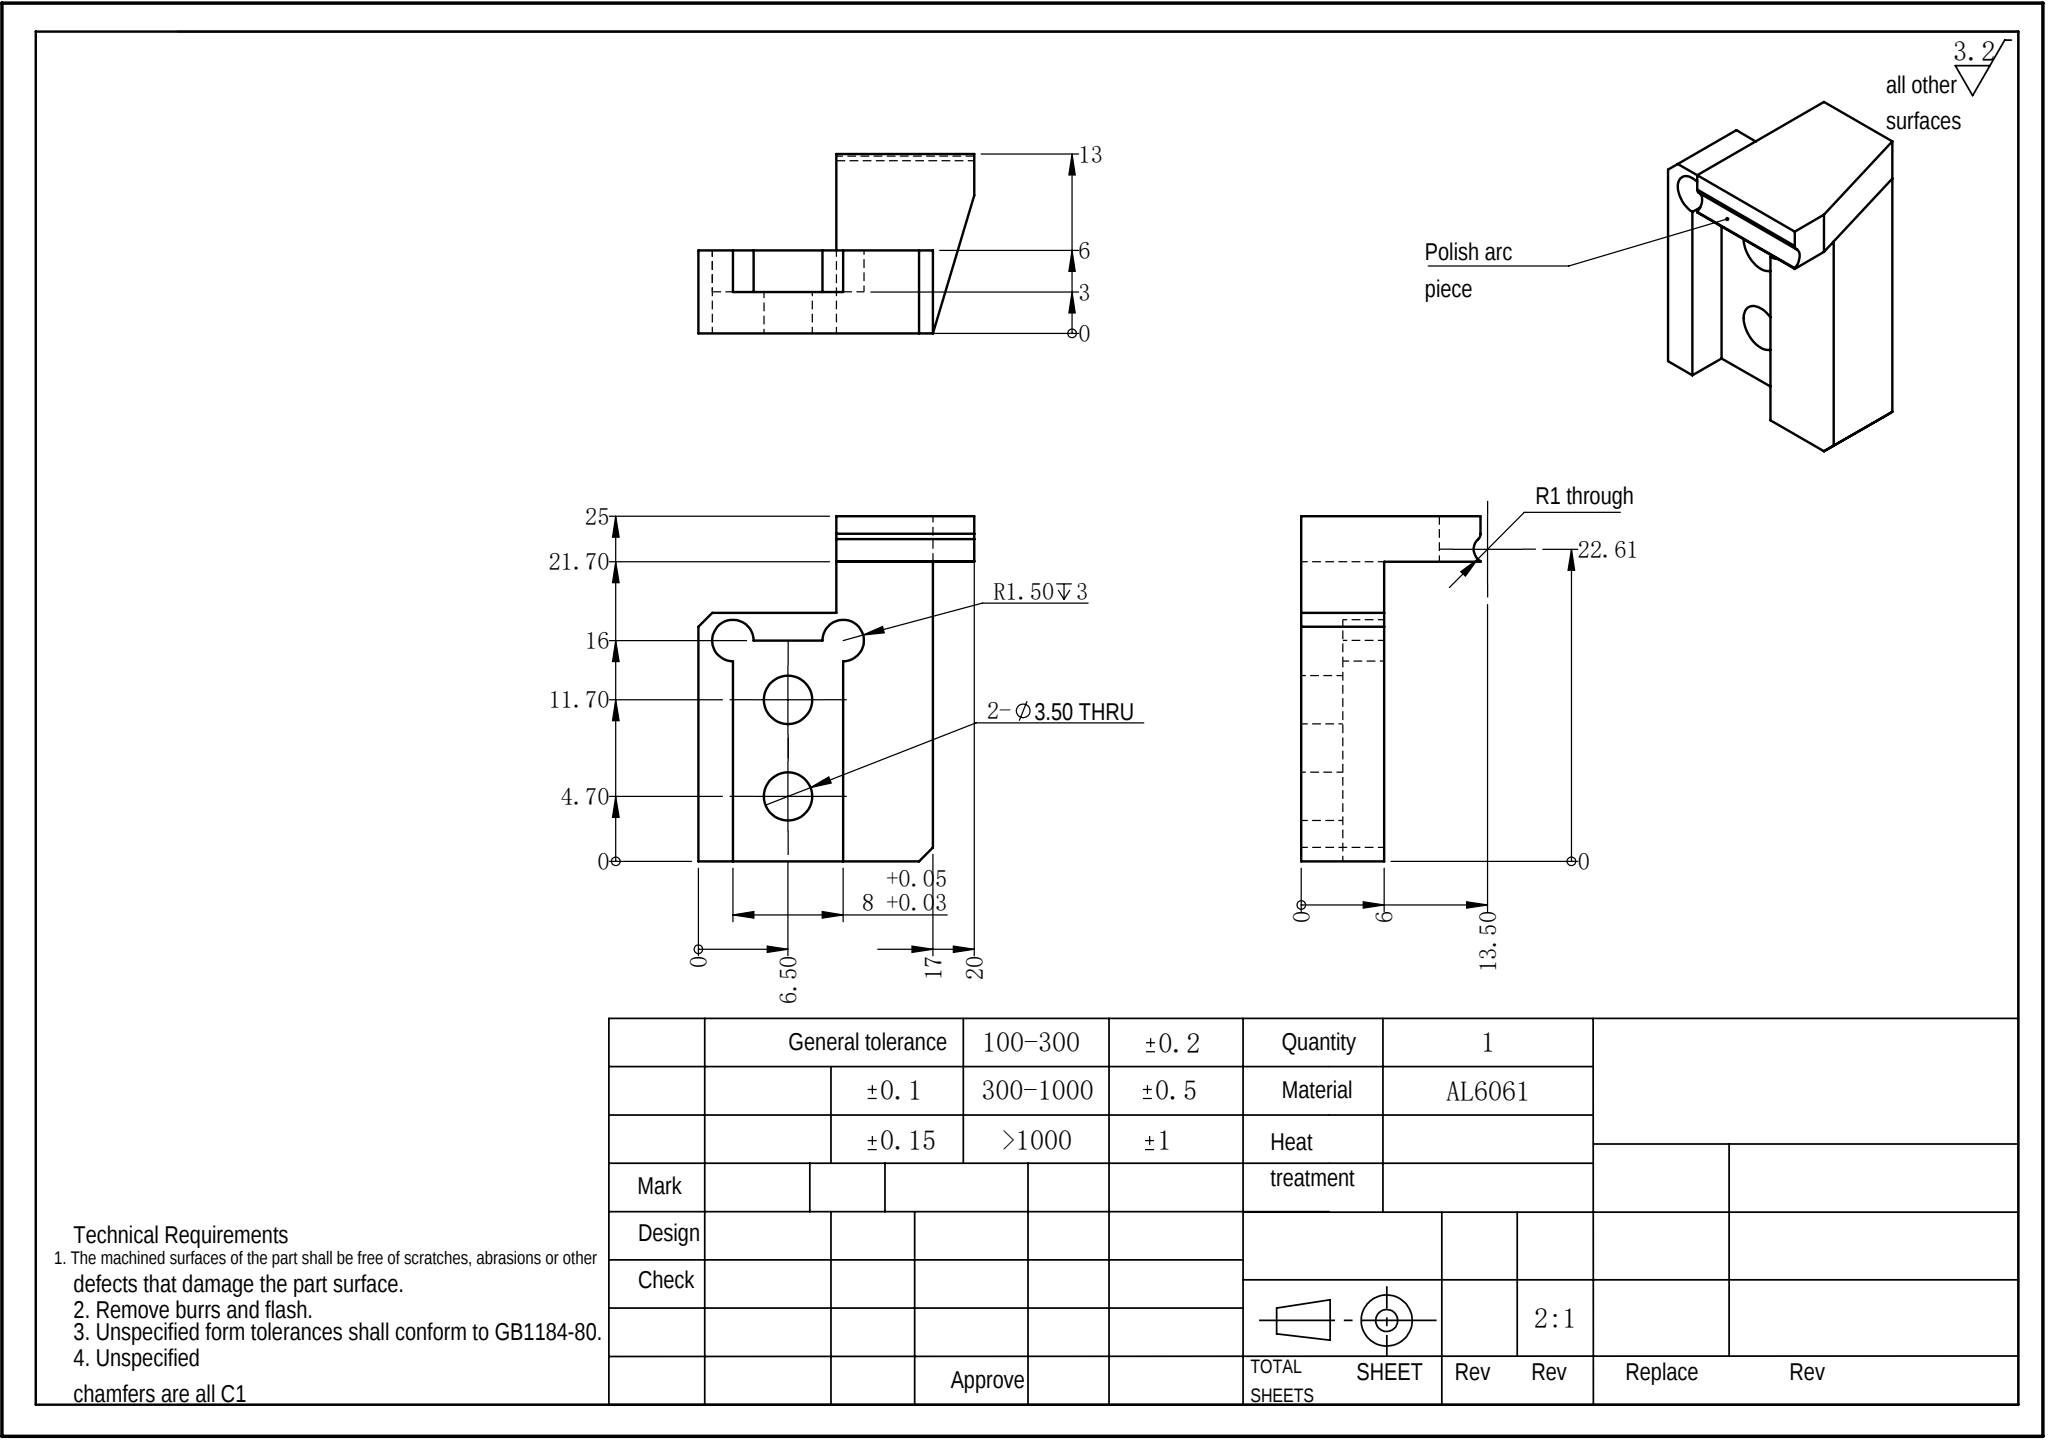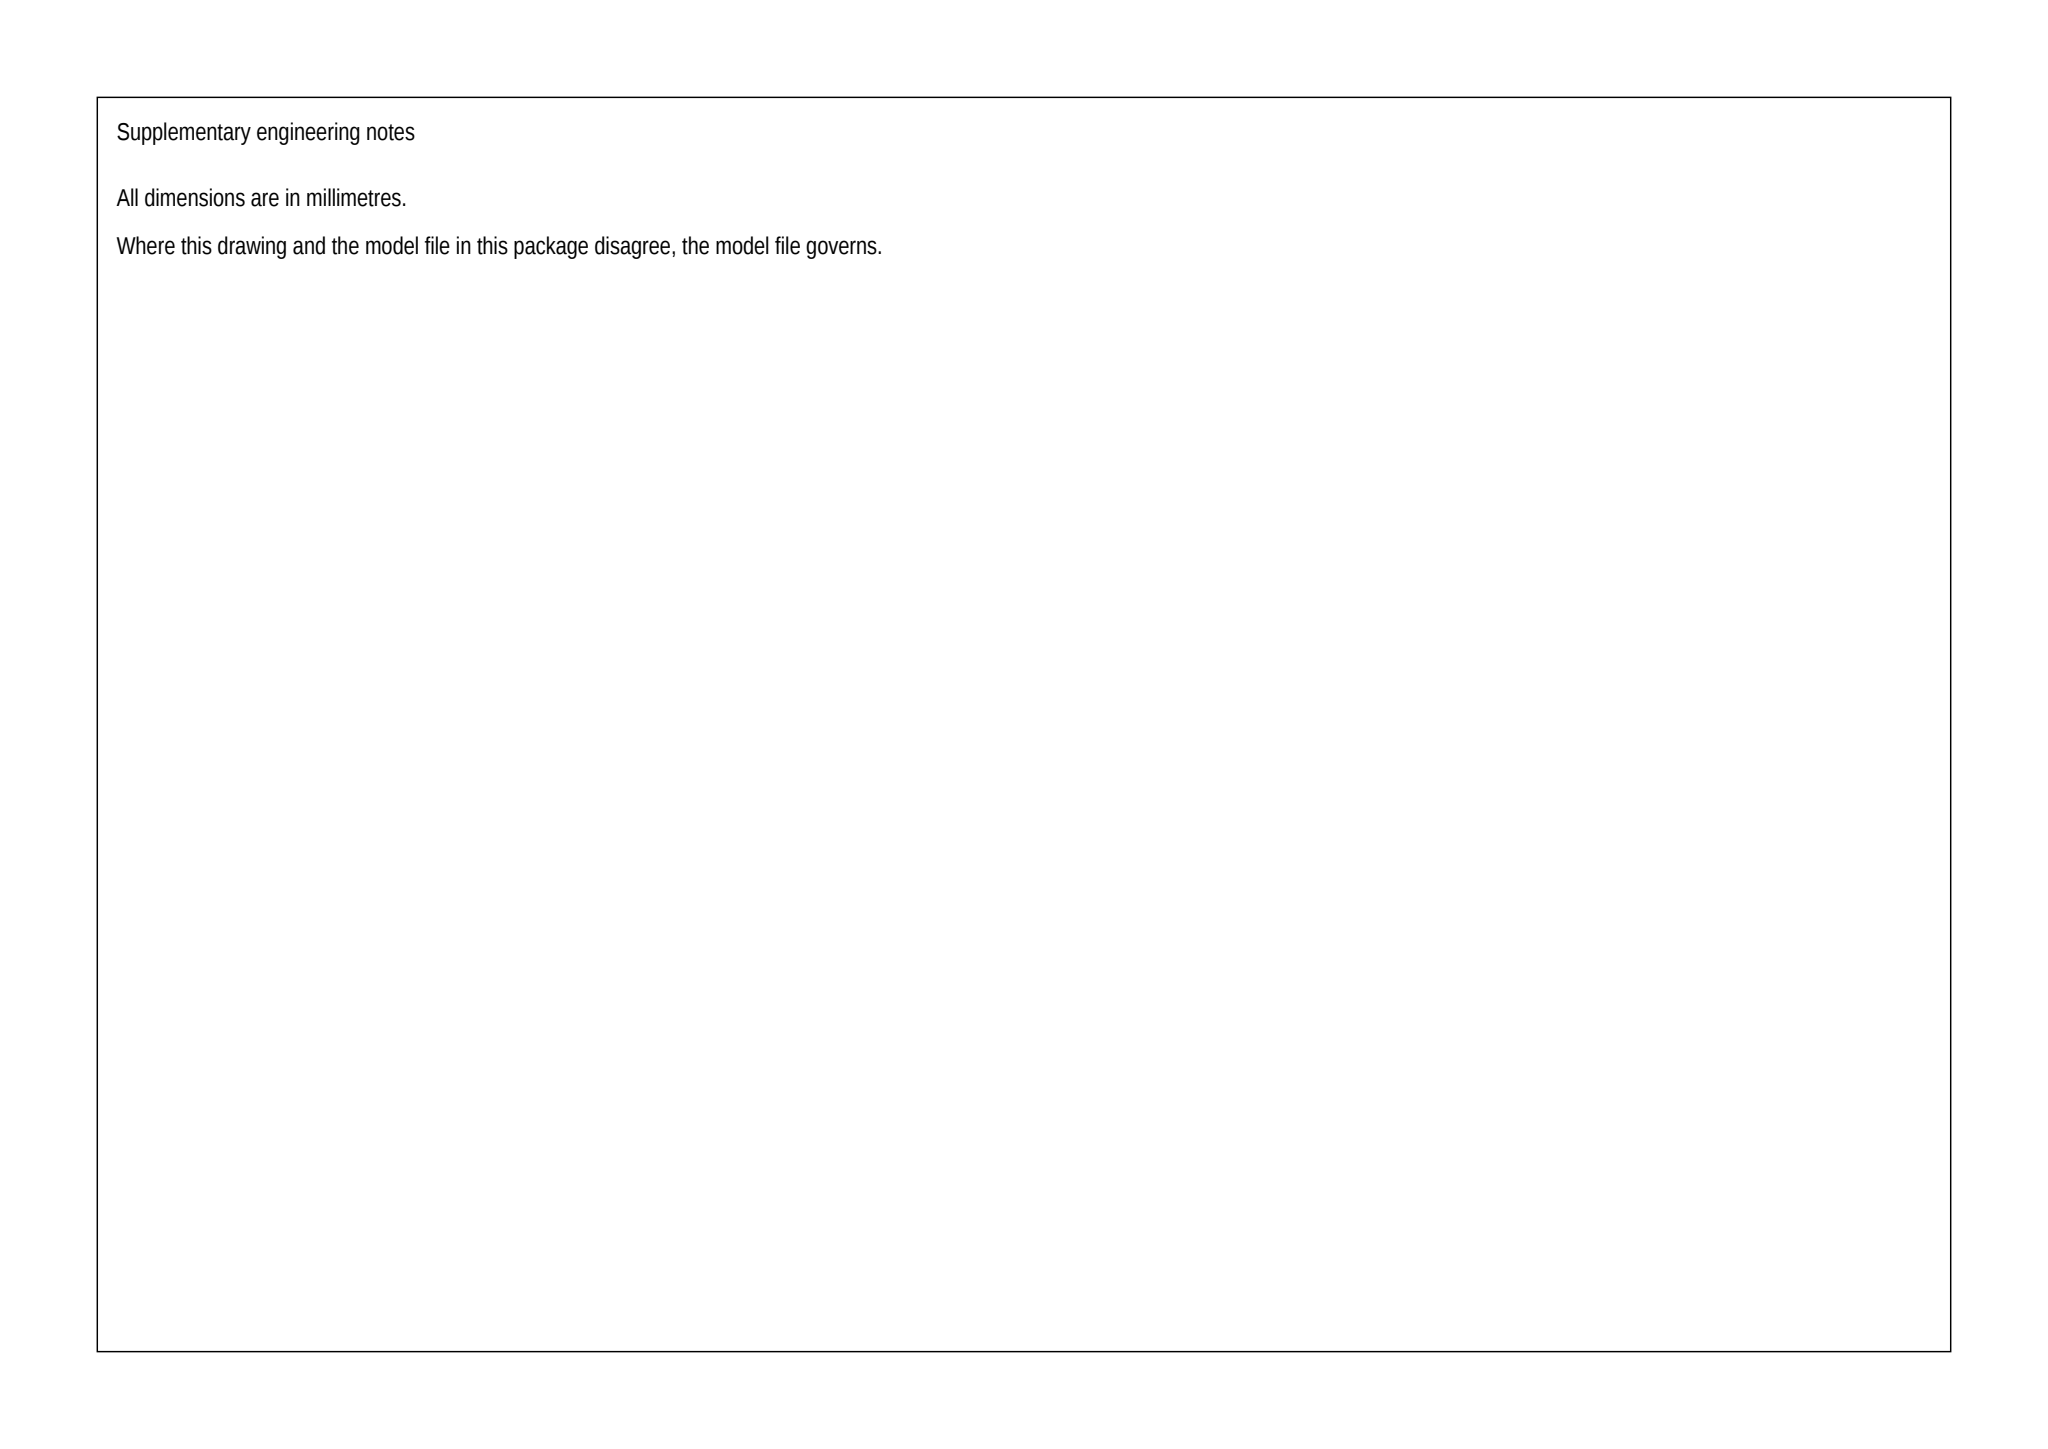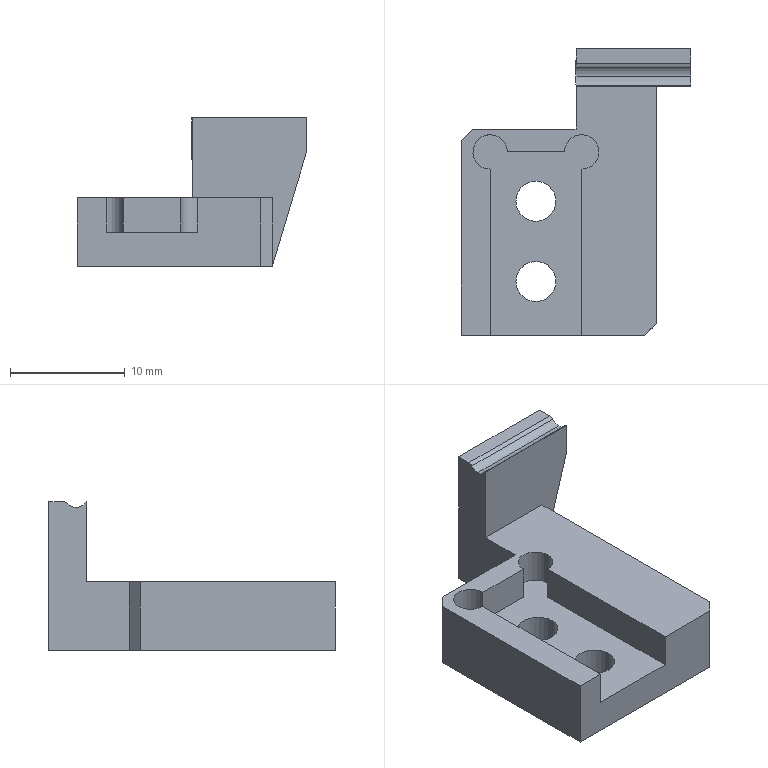Part | SolidWorks | mm | material AL6061 | 1 solid | 29 faces | box 20 x 25 x 13 mm | volume 1885 mm3 | plane 19 | cylinder 10 | commonest cylinder face diameters 3.5 x4 3 x3 2 x2 1 x1
build123d program:
from build123d import *

# Parameters (mm, degrees)
SKETCH1_W           = 20
SKETCH1_H           = 31
BOSS_EXTRUDE1_DEPTH = 12.5
SKETCH2_W           = 7
SKETCH2_H           = 18
CUT_EXTRUDE1_DEPTH  = 37
SKETCH3_W           = 19
SKETCH3_H           = 19
CUT_EXTRUDE2_DEPTH  = 37
SKETCH4_R           = 1
CUT_EXTRUDE3_DEPTH  = 37
SKETCH5_W           = 1
SKETCH5_H           = 8
CUT_EXTRUDE4_DEPTH  = 27
CHAMFER1_SIZE       = 10
CHAMFER1_SIZE2      = 3
CHAMFER2_SIZE       = 7
CHAMFER2_SIZE2      = 10
SKETCH6_W           = 21.447
SKETCH6_H           = 4.066
CUT_EXTRUDE5_DEPTH  = 10
SKETCH7_W           = 19
SKETCH7_H           = 2.7
CUT_EXTRUDE6_DEPTH  = 25
SKETCH8_W           = 8
SKETCH8_H           = 32
CUT_EXTRUDE7_DEPTH  = 3
SKETCH9_R           = 1.5
CUT_EXTRUDE8_DEPTH  = 3
SKETCH10_W          = 8
SKETCH10_H          = 32
CUT_EXTRUDE9_DEPTH  = 3
SKETCH11_R          = 1.5
CUT_EXTRUDE10_DEPTH = 3
MOVE_FACE1_BY       = 3.7
MOVE_FACE2_BY       = 3.7
SKETCH12_R          = 1.75
CUT_EXTRUDE11_DEPTH = 36
SKETCH13_W          = 42.734
SKETCH13_H          = 21.623
CUT_EXTRUDE12_DEPTH = 33
SKETCH14_W          = 10
SKETCH14_H          = 7
CUT_EXTRUDE13_DEPTH = 7
FILLET1_R           = 3
CHAMFER3_SIZE       = 7
SKETCH15_W          = 6
SKETCH15_H          = 21.7
BOSS_EXTRUDE2_DEPTH = 4
SKETCH16_W          = 13.071
SKETCH16_H          = 13.293
CUT_EXTRUDE14_DEPTH = 7
CHAMFER4_SIZE       = 1
FILLET2_R           = 0.5


with BuildPart() as part:
    # Sketch1 → Boss-Extrude1 (new, symmetric)
    with BuildSketch(Plane(origin=(0, 0, 0), x_dir=(1, 0, 0), z_dir=(0, 1, 0))):
        Rectangle(SKETCH1_W, SKETCH1_H)
    extrude(amount=BOSS_EXTRUDE1_DEPTH, both=True)

    # Sketch2 → Cut-Extrude1 (cut)
    with BuildSketch(Plane(origin=(0, 0, -15.5), x_dir=(-1, 0, 0), z_dir=(0, 0, -1))):
        with Locations((-6.5, -3.5)):
            Rectangle(SKETCH2_W, SKETCH2_H)
    extrude(amount=-CUT_EXTRUDE1_DEPTH, mode=Mode.SUBTRACT)

    # Sketch3 → Cut-Extrude2 (cut)
    with BuildSketch(Plane.ZY.offset(10)):
        with Locations((0, -3)):
            Rectangle(SKETCH3_W, SKETCH3_H)
    extrude(amount=-CUT_EXTRUDE2_DEPTH, mode=Mode.SUBTRACT)

    # Sketch4 → Cut-Extrude3 (cut)
    with BuildSketch(Plane(origin=(10, 0, 0), x_dir=(0, 0, -1), z_dir=(1, 0, 0))):
        with Locations((2, 10.11)):
            Circle(SKETCH4_R)
        with Locations((-2, 10.11)):
            Circle(SKETCH4_R)
    extrude(amount=-CUT_EXTRUDE3_DEPTH, mode=Mode.SUBTRACT)

    # Sketch5 → Cut-Extrude4 (cut)
    with BuildSketch(Plane.ZY.offset(10)):
        with Locations((2, 10.11)):
            Rectangle(SKETCH5_W, SKETCH5_H)
        with Locations((-2, 10.11)):
            Rectangle(SKETCH5_W, SKETCH5_H)
    extrude(amount=-CUT_EXTRUDE4_DEPTH, mode=Mode.SUBTRACT)


with BuildPart() as cut_extrude4_piece_1:
    # of the separate pieces the step leaves, piece 1, a body of its own (cut_extrude4_pieces)
    add(part.part.solids().sort_by_distance((-10, 12.5, -15.5))[0])

    # Chamfer1
    chamfer1_edges = [cut_extrude4_piece_1.edges().sort_by_distance(p)[0] for p in [
        (10, 9, -15.5),
    ]]
    chamfer1_side = [cut_extrude4_piece_1.faces().sort_by_distance(p)[0] for p in [
        (10, 9.244, -9.298),
    ]]
    chamfer(chamfer1_edges, length=CHAMFER1_SIZE, length2=CHAMFER1_SIZE2, reference=chamfer1_side[0])


with BuildPart() as cut_extrude4_piece_2:
    # of the separate pieces the step leaves, piece 2, a body of its own (cut_extrude4_pieces)
    add(part.part.solids().sort_by_distance((-10, 12.5, 15.5))[0])

    # Chamfer2
    chamfer2_edges = [cut_extrude4_piece_2.edges().sort_by_distance(p)[0] for p in [
        (10, 9, 15.5),
    ]]
    chamfer2_side = [cut_extrude4_piece_2.faces().sort_by_distance(p)[0] for p in [
        (-2.19, 1.179, 15.5),
    ]]
    chamfer(chamfer2_edges, length=CHAMFER2_SIZE, length2=CHAMFER2_SIZE2, reference=chamfer2_side[0])


with BuildPart() as cut_extrude4_piece_3:
    # of the separate pieces the step leaves, piece 3, a body of its own (cut_extrude4_pieces)
    add(part.part.solids().sort_by_distance((-10, 12.5, -1.5))[0])

    # Sketch6 → Cut-Extrude5 (cut)
    with BuildSketch(Plane(origin=(0, 12.5, 0), x_dir=(1, 0, 0), z_dir=(0, 1, 0))):
        with Locations((0.1463, 0.06726)):
            Rectangle(SKETCH6_W, SKETCH6_H)
    extrude(amount=-CUT_EXTRUDE5_DEPTH, mode=Mode.SUBTRACT)


with BuildPart() as cut_extrude6_tool:
    # Sketch7 → Cut-Extrude6 (new body)
    with BuildSketch(Plane.ZY.offset(10)):
        with Locations((0, 7.85)):
            Rectangle(SKETCH7_W, SKETCH7_H)
    extrude(amount=-CUT_EXTRUDE6_DEPTH)


with BuildPart() as cut_extrude4_piece_1_1:
    add(cut_extrude4_piece_1.part)

    # Cut-Extrude6: cut by cut_extrude6_tool
    add(cut_extrude6_tool.part, mode=Mode.SUBTRACT)

    # Sketch8 → Cut-Extrude7 (cut)
    with BuildSketch(Plane.XY.offset(-9.5)):
        with Locations((-3.5, -12.5)):
            Rectangle(SKETCH8_W, SKETCH8_H)
    extrude(amount=-CUT_EXTRUDE7_DEPTH, mode=Mode.SUBTRACT)

    # Sketch9 → Cut-Extrude8 (cut)
    with BuildSketch(Plane.XY.offset(-9.5)):
        with Locations((0.5, 3.5)):
            Circle(SKETCH9_R)
        with Locations((-7.5, 3.5)):
            Circle(SKETCH9_R)
    extrude(amount=-CUT_EXTRUDE8_DEPTH, mode=Mode.SUBTRACT)

    # Move Face1: a face moved inward by 3.7
    extrude(cut_extrude4_piece_1_1.faces().sort_by_distance((5.478, 5.5, -12.316))[0], amount=MOVE_FACE1_BY, dir=(0, 1, 0), mode=Mode.SUBTRACT)


with BuildPart() as cut_extrude4_piece_2_1:
    add(cut_extrude4_piece_2.part)

    # Cut-Extrude6: cut by cut_extrude6_tool
    add(cut_extrude6_tool.part, mode=Mode.SUBTRACT)

    # Sketch10 → Cut-Extrude9 (cut)
    with BuildSketch(Plane(origin=(0, 0, 9.5), x_dir=(-1, 0, 0), z_dir=(0, 0, -1))):
        with Locations((3.5, -12.5)):
            Rectangle(SKETCH10_W, SKETCH10_H)
    extrude(amount=-CUT_EXTRUDE9_DEPTH, mode=Mode.SUBTRACT)

    # Sketch11 → Cut-Extrude10 (cut)
    with BuildSketch(Plane(origin=(0, 0, 9.5), x_dir=(-1, 0, 0), z_dir=(0, 0, -1))):
        with Locations((7.5, 3.5)):
            Circle(SKETCH11_R)
        with Locations((-0.5, 3.5)):
            Circle(SKETCH11_R)
    extrude(amount=-CUT_EXTRUDE10_DEPTH, mode=Mode.SUBTRACT)

    # Move Face2: a face moved inward by 3.7
    extrude(cut_extrude4_piece_2_1.faces().sort_by_distance((4.4, 5.5, 11.5))[0], amount=MOVE_FACE2_BY, dir=(0, 1, 0), mode=Mode.SUBTRACT)


with BuildPart() as cut_extrude11_tool:
    # Sketch12 → Cut-Extrude11 (new body)
    with BuildSketch(Plane.XY.offset(15.5)):
        with Locations((-3.5, -0.8)):
            Circle(SKETCH12_R)
        with Locations((-3.5, -7.8)):
            Circle(SKETCH12_R)
    extrude(amount=-CUT_EXTRUDE11_DEPTH)


with BuildPart() as cut_extrude4_piece_1_2:
    add(cut_extrude4_piece_1_1.part)

    # Cut-Extrude11: cut by cut_extrude11_tool
    add(cut_extrude11_tool.part, mode=Mode.SUBTRACT)

    # Sketch14 → Cut-Extrude13 (cut)
    with BuildSketch(Plane.XZ.offset(-9.2)):
        with Locations((-5, -6)):
            Rectangle(SKETCH14_W, SKETCH14_H)
    extrude(amount=-CUT_EXTRUDE13_DEPTH, mode=Mode.SUBTRACT)

    # Fillet1
    fillet1_edges = [cut_extrude4_piece_1_2.edges().sort_by_distance(p)[0] for p in [
        (0, 10.85, -9.5),
    ]]
    fillet(fillet1_edges, radius=FILLET1_R)

    # Chamfer3
    chamfer3_edges = [cut_extrude4_piece_1_2.edges().sort_by_distance(p)[0] for p in [
        (-10, 12.5, -12.5),
    ]]
    chamfer(chamfer3_edges, length=CHAMFER3_SIZE)

    # Sketch15 → Boss-Extrude2 (add)
    with BuildSketch(Plane(origin=(3, 0, 0), x_dir=(0, 0, -1), z_dir=(1, 0, 0))):
        with Locations((12.5, -1.65)):
            Rectangle(SKETCH15_W, SKETCH15_H)
    extrude(amount=BOSS_EXTRUDE2_DEPTH)

    # Sketch16 → Cut-Extrude14 (cut)
    with BuildSketch(Plane(origin=(0, 12.5, 0), x_dir=(1, 0, 0), z_dir=(0, 1, 0))):
        with Locations((-6.536, 11.307)):
            Rectangle(SKETCH16_W, SKETCH16_H)
    extrude(amount=-CUT_EXTRUDE14_DEPTH, mode=Mode.SUBTRACT)

    # Chamfer4
    chamfer4_edges = [cut_extrude4_piece_1_2.edges().sort_by_distance(p)[0] for p in [
        (-10, 5.5, -12.5),
        (7, -12.5, -12.5),
    ]]
    chamfer(chamfer4_edges, length=CHAMFER4_SIZE)

    # Fillet2
    fillet2_edges = [cut_extrude4_piece_1_2.edges().sort_by_distance(p)[0] for p in [
        (5, 10.976, -2.5),
    ]]
    fillet(fillet2_edges, radius=FILLET2_R)


with BuildPart() as cut_extrude4_piece_2_2:
    add(cut_extrude4_piece_2_1.part)

    # Cut-Extrude11: cut by cut_extrude11_tool
    add(cut_extrude11_tool.part, mode=Mode.SUBTRACT)

    # Sketch13 → Cut-Extrude12 (cut)
    with BuildSketch(Plane(origin=(0, 12.5, 0), x_dir=(1, 0, 0), z_dir=(0, 1, 0))):
        with Locations((-1.795, -10.299)):
            Rectangle(SKETCH13_W, SKETCH13_H)
    extrude(amount=-CUT_EXTRUDE12_DEPTH, mode=Mode.SUBTRACT)


solid = cut_extrude4_piece_1_2.part